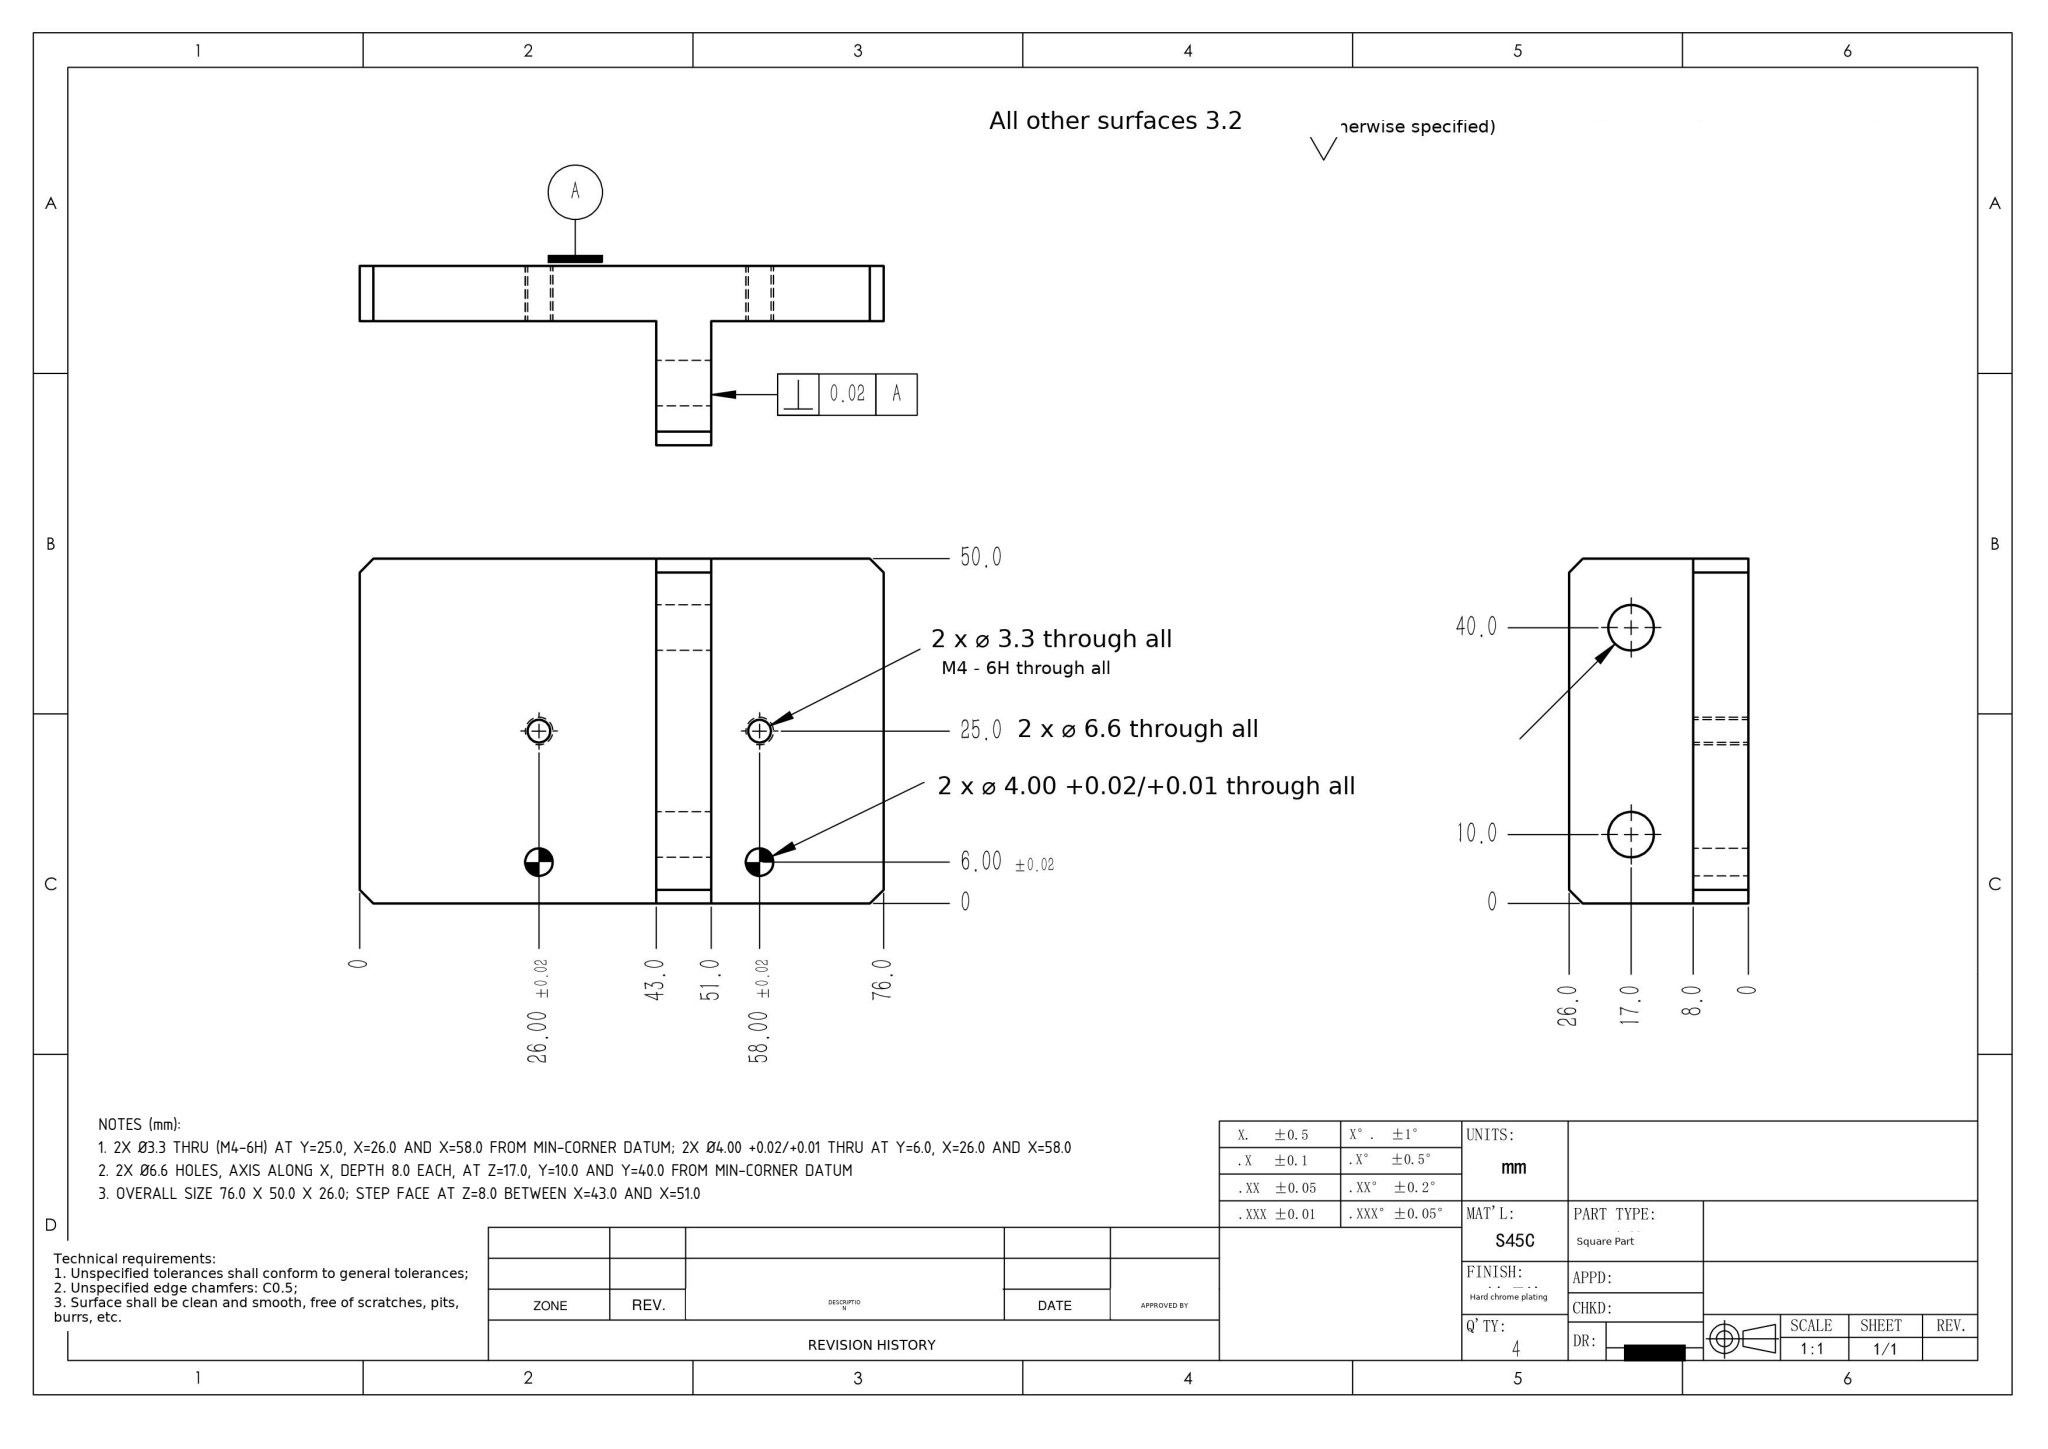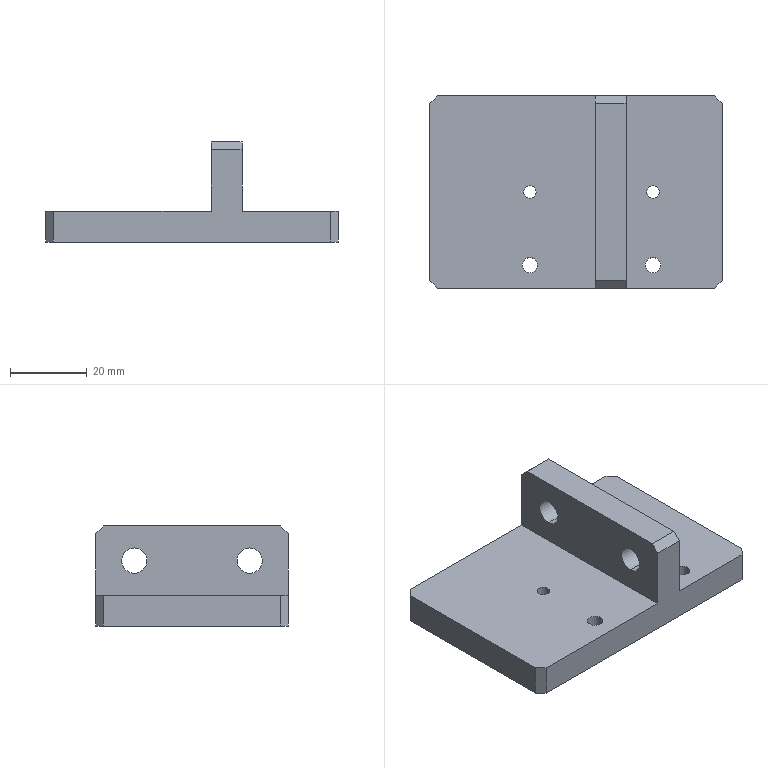Part | SolidWorks | mm | 1 solid | 28 faces | box 76 x 50 x 26 mm | volume 36619 mm3 | plane 16 | cylinder 12 | commonest cylinder face diameters 6.6 x4 4 x4 3.3 x4
Drawing notes:
2X Ø3.3 THRU (M4-6H) AT Y=25.0, X=26.0 AND X=58.0 FROM MIN-CORNER DATUM; 2X Ø4.00 +0.02/+0.01 THRU AT Y=6.0, X=26.0 AND X=58.0 | from the solid: cylinders dia 3.3 axis z at (26,25) and (58,25); dia 4.0 axis z at (26,6) and (58,6)
2X Ø6.6 HOLES, AXIS ALONG X, DEPTH 8.0 EACH, AT Z=17.0, Y=10.0 AND Y=40.0 FROM MIN-CORNER DATUM | from the solid: cylinders dia 6.6 axis x, pos (y=10,z=17) and (y=40,z=17), length 8.0
OVERALL SIZE 76.0 X 50.0 X 26.0; STEP FACE AT Z=8.0 BETWEEN X=43.0 AND X=51.0 | from the solid: bbox_xyz 76/50/26; axis_planes z=8.0 (2), x=43.0, x=51.0
build123d program:
from build123d import *

# Parameters (mm, degrees)
SKETCH1_W                 = 76
SKETCH1_H                 = 50
BOSS_EXTRUDE1_DEPTH       = 8
SKETCH2_W                 = 8
SKETCH2_H                 = 50
BOSS_EXTRUDE2_DEPTH       = 18
M4_TAPPED_HOLE1_D         = 3.3
SIZE_MM_DOWEL_PIN_HOLE1_D = 4
M6_CLEARANCE_HOLE1_D      = 6.6
CHAMFER1_SIZE             = 2


with BuildPart() as part:
    # Sketch1 → Boss-Extrude1 (new body)
    with BuildSketch(Plane.XY):
        Rectangle(SKETCH1_W, SKETCH1_H)
    extrude(amount=BOSS_EXTRUDE1_DEPTH)

    # Sketch2 → Boss-Extrude2 (add)
    with BuildSketch(Plane.XY.offset(8)):
        with Locations((9, 0)):
            Rectangle(SKETCH2_W, SKETCH2_H)
    extrude(amount=BOSS_EXTRUDE2_DEPTH)

    # M4 Tapped Hole1 (through all)
    with Locations(Plane.XY.offset(8)):
        with Locations((-12, 0), (20, 0)):
            Hole(M4_TAPPED_HOLE1_D / 2)

    # Size mm Dowel Pin Hole1 (through all)
    with Locations(Plane(origin=(0, 0, 0), x_dir=(1, 0, 0), z_dir=(0, 0, -1))):
        with Locations((-12, 19), (20, 19)):
            Hole(SIZE_MM_DOWEL_PIN_HOLE1_D / 2)

    # M6 Clearance Hole1 (through all)
    with Locations(Plane(origin=(13, 0, 0), x_dir=(0, 0, -1), z_dir=(1, 0, 0))):
        with Locations((-17, 15), (-17, -15)):
            Hole(M6_CLEARANCE_HOLE1_D / 2)

    # Chamfer1
    chamfer1_edges = [part.edges().sort_by_distance(p)[0] for p in [
        (9, -25, 26),
        (9, 25, 26),
        (38, -25, 4),
        (-38, -25, 4),
        (-38, 25, 4),
        (38, 25, 4),
    ]]
    chamfer(chamfer1_edges, length=CHAMFER1_SIZE)


solid = part.part
STEP:
#1=CARTESIAN_POINT('',(5.,15.,20.3));
#2=VERTEX_POINT('',#1);
#3=CARTESIAN_POINT('',(5.,15.,13.7));
#4=VERTEX_POINT('',#3);
#5=CARTESIAN_POINT('',(5.,15.,17.));
#6=DIRECTION('',(1.,0.,0.));
#7=DIRECTION('',(0.,1.,0.));
#8=AXIS2_PLACEMENT_3D('',#5,#6,#7);
#9=CIRCLE('',#8,3.3);
#10=EDGE_CURVE('',#2,#4,#9,.T.);
#11=ORIENTED_EDGE('',*,*,#10,.F.);
#12=CARTESIAN_POINT('',(13.,15.,20.3));
#13=VERTEX_POINT('',#12);
#14=CARTESIAN_POINT('',(13.,15.,20.3));
#15=DIRECTION('',(1.,0.,0.));
#16=VECTOR('',#15,1000.);
#17=LINE('',#14,#16);
#18=EDGE_CURVE('',#2,#13,#17,.T.);
#19=ORIENTED_EDGE('',*,*,#18,.T.);
#20=CARTESIAN_POINT('',(13.,15.,13.7));
#21=VERTEX_POINT('',#20);
#22=CARTESIAN_POINT('',(13.,15.,17.));
#23=DIRECTION('',(1.,0.,0.));
#24=DIRECTION('',(0.,0.,-1.));
#25=AXIS2_PLACEMENT_3D('',#22,#23,#24);
#26=CIRCLE('',#25,3.3);
#27=EDGE_CURVE('',#13,#21,#26,.T.);
#28=ORIENTED_EDGE('',*,*,#27,.T.);
#29=CARTESIAN_POINT('',(13.,15.,13.7));
#30=DIRECTION('',(1.,0.,0.));
#31=VECTOR('',#30,1000.);
#32=LINE('',#29,#31);
#33=EDGE_CURVE('',#4,#21,#32,.T.);
#34=ORIENTED_EDGE('',*,*,#33,.F.);
#35=EDGE_LOOP('',(#11,#19,#28,#34));
#36=FACE_OUTER_BOUND('',#35,.T.);
#37=CARTESIAN_POINT('',(13.,15.,17.));
#38=DIRECTION('',(1.,0.,0.));
#39=DIRECTION('',(0.,0.,-1.));
#40=AXIS2_PLACEMENT_3D('',#37,#38,#39);
#41=CYLINDRICAL_SURFACE('',#40,3.3);
#42=ADVANCED_FACE('',(#36),#41,.F.);
#43=CARTESIAN_POINT('',(5.,-15.,20.3));
#44=VERTEX_POINT('',#43);
#45=CARTESIAN_POINT('',(5.,-15.,13.7));
#46=VERTEX_POINT('',#45);
#47=CARTESIAN_POINT('',(5.,-15.,17.));
#48=DIRECTION('',(1.,0.,0.));
#49=DIRECTION('',(0.,1.,0.));
#50=AXIS2_PLACEMENT_3D('',#47,#48,#49);
#51=CIRCLE('',#50,3.3);
#52=EDGE_CURVE('',#44,#46,#51,.T.);
#53=ORIENTED_EDGE('',*,*,#52,.F.);
#54=CARTESIAN_POINT('',(13.,-15.,20.3));
#55=VERTEX_POINT('',#54);
#56=CARTESIAN_POINT('',(13.,-15.,20.3));
#57=DIRECTION('',(1.,0.,0.));
#58=VECTOR('',#57,1000.);
#59=LINE('',#56,#58);
#60=EDGE_CURVE('',#44,#55,#59,.T.);
#61=ORIENTED_EDGE('',*,*,#60,.T.);
#62=CARTESIAN_POINT('',(13.,-15.,13.7));
#63=VERTEX_POINT('',#62);
#64=CARTESIAN_POINT('',(13.,-15.,17.));
#65=DIRECTION('',(1.,0.,0.));
#66=DIRECTION('',(0.,0.,-1.));
#67=AXIS2_PLACEMENT_3D('',#64,#65,#66);
#68=CIRCLE('',#67,3.3);
#69=EDGE_CURVE('',#55,#63,#68,.T.);
#70=ORIENTED_EDGE('',*,*,#69,.T.);
#71=CARTESIAN_POINT('',(13.,-15.,13.7));
#72=DIRECTION('',(1.,0.,0.));
#73=VECTOR('',#72,1000.);
#74=LINE('',#71,#73);
#75=EDGE_CURVE('',#46,#63,#74,.T.);
#76=ORIENTED_EDGE('',*,*,#75,.F.);
#77=EDGE_LOOP('',(#53,#61,#70,#76));
#78=FACE_OUTER_BOUND('',#77,.T.);
#79=CARTESIAN_POINT('',(13.,-15.,17.));
#80=DIRECTION('',(1.,0.,0.));
#81=DIRECTION('',(0.,0.,-1.));
#82=AXIS2_PLACEMENT_3D('',#79,#80,#81);
#83=CYLINDRICAL_SURFACE('',#82,3.3);
#84=ADVANCED_FACE('',(#78),#83,.F.);
#85=CARTESIAN_POINT('',(-14.,-19.,8.));
#86=VERTEX_POINT('',#85);
#87=CARTESIAN_POINT('',(-10.,-19.,8.));
#88=VERTEX_POINT('',#87);
#89=CARTESIAN_POINT('',(-12.,-19.,8.));
#90=DIRECTION('',(0.,0.,1.));
#91=DIRECTION('',(1.,0.,0.));
#92=AXIS2_PLACEMENT_3D('',#89,#90,#91);
#93=CIRCLE('',#92,2.);
#94=EDGE_CURVE('',#86,#88,#93,.T.);
#95=ORIENTED_EDGE('',*,*,#94,.T.);
#96=CARTESIAN_POINT('',(-10.,-19.,0.));
#97=VERTEX_POINT('',#96);
#98=CARTESIAN_POINT('',(-10.,-19.,0.));
#99=DIRECTION('',(0.,0.,-1.));
#100=VECTOR('',#99,1000.);
#101=LINE('',#98,#100);
#102=EDGE_CURVE('',#88,#97,#101,.T.);
#103=ORIENTED_EDGE('',*,*,#102,.T.);
#104=CARTESIAN_POINT('',(-14.,-19.,0.));
#105=VERTEX_POINT('',#104);
#106=CARTESIAN_POINT('',(-12.,-19.,0.));
#107=DIRECTION('',(0.,0.,-1.));
#108=DIRECTION('',(-1.,0.,0.));
#109=AXIS2_PLACEMENT_3D('',#106,#107,#108);
#110=CIRCLE('',#109,2.);
#111=EDGE_CURVE('',#97,#105,#110,.T.);
#112=ORIENTED_EDGE('',*,*,#111,.T.);
#113=CARTESIAN_POINT('',(-14.,-19.,0.));
#114=DIRECTION('',(0.,0.,-1.));
#115=VECTOR('',#114,1000.);
#116=LINE('',#113,#115);
#117=EDGE_CURVE('',#86,#105,#116,.T.);
#118=ORIENTED_EDGE('',*,*,#117,.F.);
#119=EDGE_LOOP('',(#95,#103,#112,#118));
#120=FACE_OUTER_BOUND('',#119,.T.);
#121=CARTESIAN_POINT('',(-12.,-19.,0.));
#122=DIRECTION('',(0.,0.,-1.));
#123=DIRECTION('',(-1.,0.,0.));
#124=AXIS2_PLACEMENT_3D('',#121,#122,#123);
#125=CYLINDRICAL_SURFACE('',#124,2.);
#126=ADVANCED_FACE('',(#120),#125,.F.);
#127=CARTESIAN_POINT('',(18.,-19.,8.));
#128=VERTEX_POINT('',#127);
#129=CARTESIAN_POINT('',(22.,-19.,8.));
#130=VERTEX_POINT('',#129);
#131=CARTESIAN_POINT('',(20.,-19.,8.));
#132=DIRECTION('',(0.,0.,1.));
#133=DIRECTION('',(1.,0.,0.));
#134=AXIS2_PLACEMENT_3D('',#131,#132,#133);
#135=CIRCLE('',#134,2.);
#136=EDGE_CURVE('',#128,#130,#135,.T.);
#137=ORIENTED_EDGE('',*,*,#136,.T.);
#138=CARTESIAN_POINT('',(22.,-19.,0.));
#139=VERTEX_POINT('',#138);
#140=CARTESIAN_POINT('',(22.,-19.,0.));
#141=DIRECTION('',(0.,0.,-1.));
#142=VECTOR('',#141,1000.);
#143=LINE('',#140,#142);
#144=EDGE_CURVE('',#130,#139,#143,.T.);
#145=ORIENTED_EDGE('',*,*,#144,.T.);
#146=CARTESIAN_POINT('',(18.,-19.,0.));
#147=VERTEX_POINT('',#146);
#148=CARTESIAN_POINT('',(20.,-19.,0.));
#149=DIRECTION('',(0.,0.,-1.));
#150=DIRECTION('',(-1.,0.,0.));
#151=AXIS2_PLACEMENT_3D('',#148,#149,#150);
#152=CIRCLE('',#151,2.);
#153=EDGE_CURVE('',#139,#147,#152,.T.);
#154=ORIENTED_EDGE('',*,*,#153,.T.);
#155=CARTESIAN_POINT('',(18.,-19.,0.));
#156=DIRECTION('',(0.,0.,-1.));
#157=VECTOR('',#156,1000.);
#158=LINE('',#155,#157);
#159=EDGE_CURVE('',#128,#147,#158,.T.);
#160=ORIENTED_EDGE('',*,*,#159,.F.);
#161=EDGE_LOOP('',(#137,#145,#154,#160));
#162=FACE_OUTER_BOUND('',#161,.T.);
#163=CARTESIAN_POINT('',(20.,-19.,0.));
#164=DIRECTION('',(0.,0.,-1.));
#165=DIRECTION('',(-1.,0.,0.));
#166=AXIS2_PLACEMENT_3D('',#163,#164,#165);
#167=CYLINDRICAL_SURFACE('',#166,2.);
#168=ADVANCED_FACE('',(#162),#167,.F.);
#169=CARTESIAN_POINT('',(-13.65,0.,0.));
#170=VERTEX_POINT('',#169);
#171=CARTESIAN_POINT('',(-10.35,0.,0.));
#172=VERTEX_POINT('',#171);
#173=CARTESIAN_POINT('',(-12.,0.,0.));
#174=DIRECTION('',(0.,0.,1.));
#175=DIRECTION('',(1.,0.,0.));
#176=AXIS2_PLACEMENT_3D('',#173,#174,#175);
#177=CIRCLE('',#176,1.65);
#178=EDGE_CURVE('',#170,#172,#177,.T.);
#179=ORIENTED_EDGE('',*,*,#178,.F.);
#180=CARTESIAN_POINT('',(-13.65,0.,8.));
#181=VERTEX_POINT('',#180);
#182=CARTESIAN_POINT('',(-13.65,0.,8.));
#183=DIRECTION('',(0.,0.,1.));
#184=VECTOR('',#183,1000.);
#185=LINE('',#182,#184);
#186=EDGE_CURVE('',#170,#181,#185,.T.);
#187=ORIENTED_EDGE('',*,*,#186,.T.);
#188=CARTESIAN_POINT('',(-10.35,0.,8.));
#189=VERTEX_POINT('',#188);
#190=CARTESIAN_POINT('',(-12.,0.,8.));
#191=DIRECTION('',(0.,0.,1.));
#192=DIRECTION('',(1.,0.,0.));
#193=AXIS2_PLACEMENT_3D('',#190,#191,#192);
#194=CIRCLE('',#193,1.65);
#195=EDGE_CURVE('',#181,#189,#194,.T.);
#196=ORIENTED_EDGE('',*,*,#195,.T.);
#197=CARTESIAN_POINT('',(-10.35,0.,8.));
#198=DIRECTION('',(0.,0.,1.));
#199=VECTOR('',#198,1000.);
#200=LINE('',#197,#199);
#201=EDGE_CURVE('',#172,#189,#200,.T.);
#202=ORIENTED_EDGE('',*,*,#201,.F.);
#203=EDGE_LOOP('',(#179,#187,#196,#202));
#204=FACE_OUTER_BOUND('',#203,.T.);
#205=CARTESIAN_POINT('',(-12.,0.,8.));
#206=DIRECTION('',(0.,0.,1.));
#207=DIRECTION('',(1.,0.,0.));
#208=AXIS2_PLACEMENT_3D('',#205,#206,#207);
#209=CYLINDRICAL_SURFACE('',#208,1.65);
#210=ADVANCED_FACE('',(#204),#209,.F.);
#211=CARTESIAN_POINT('',(18.35,0.,0.));
#212=VERTEX_POINT('',#211);
#213=CARTESIAN_POINT('',(21.65,0.,0.));
#214=VERTEX_POINT('',#213);
#215=CARTESIAN_POINT('',(20.,0.,0.));
#216=DIRECTION('',(0.,0.,1.));
#217=DIRECTION('',(1.,0.,0.));
#218=AXIS2_PLACEMENT_3D('',#215,#216,#217);
#219=CIRCLE('',#218,1.65);
#220=EDGE_CURVE('',#212,#214,#219,.T.);
#221=ORIENTED_EDGE('',*,*,#220,.F.);
#222=CARTESIAN_POINT('',(18.35,0.,8.));
#223=VERTEX_POINT('',#222);
#224=CARTESIAN_POINT('',(18.35,0.,8.));
#225=DIRECTION('',(0.,0.,1.));
#226=VECTOR('',#225,1000.);
#227=LINE('',#224,#226);
#228=EDGE_CURVE('',#212,#223,#227,.T.);
#229=ORIENTED_EDGE('',*,*,#228,.T.);
#230=CARTESIAN_POINT('',(21.65,0.,8.));
#231=VERTEX_POINT('',#230);
#232=CARTESIAN_POINT('',(20.,0.,8.));
#233=DIRECTION('',(0.,0.,1.));
#234=DIRECTION('',(1.,0.,0.));
#235=AXIS2_PLACEMENT_3D('',#232,#233,#234);
#236=CIRCLE('',#235,1.65);
#237=EDGE_CURVE('',#223,#231,#236,.T.);
#238=ORIENTED_EDGE('',*,*,#237,.T.);
#239=CARTESIAN_POINT('',(21.65,0.,8.));
#240=DIRECTION('',(0.,0.,1.));
#241=VECTOR('',#240,1000.);
#242=LINE('',#239,#241);
#243=EDGE_CURVE('',#214,#231,#242,.T.);
#244=ORIENTED_EDGE('',*,*,#243,.F.);
#245=EDGE_LOOP('',(#221,#229,#238,#244));
#246=FACE_OUTER_BOUND('',#245,.T.);
#247=CARTESIAN_POINT('',(20.,0.,8.));
#248=DIRECTION('',(0.,0.,1.));
#249=DIRECTION('',(1.,0.,0.));
#250=AXIS2_PLACEMENT_3D('',#247,#248,#249);
#251=CYLINDRICAL_SURFACE('',#250,1.65);
#252=ADVANCED_FACE('',(#246),#251,.F.);
#253=ORIENTED_EDGE('',*,*,#94,.F.);
#254=CARTESIAN_POINT('',(-12.,-19.,8.));
#255=DIRECTION('',(0.,0.,1.));
#256=DIRECTION('',(1.,0.,0.));
#257=AXIS2_PLACEMENT_3D('',#254,#255,#256);
#258=CIRCLE('',#257,2.);
#259=EDGE_CURVE('',#88,#86,#258,.T.);
#260=ORIENTED_EDGE('',*,*,#259,.F.);
#261=EDGE_LOOP('',(#253,#260));
#262=FACE_BOUND('',#261,.T.);
#263=CARTESIAN_POINT('',(-12.,0.,8.));
#264=DIRECTION('',(0.,0.,1.));
#265=DIRECTION('',(1.,0.,0.));
#266=AXIS2_PLACEMENT_3D('',#263,#264,#265);
#267=CIRCLE('',#266,1.65);
#268=EDGE_CURVE('',#189,#181,#267,.T.);
#269=ORIENTED_EDGE('',*,*,#268,.F.);
#270=ORIENTED_EDGE('',*,*,#195,.F.);
#271=EDGE_LOOP('',(#269,#270));
#272=FACE_BOUND('',#271,.T.);
#273=CARTESIAN_POINT('',(5.,25.,8.));
#274=VERTEX_POINT('',#273);
#275=CARTESIAN_POINT('',(-36.,25.,8.));
#276=VERTEX_POINT('',#275);
#277=CARTESIAN_POINT('',(-38.,25.,8.));
#278=DIRECTION('',(-1.,0.,0.));
#279=VECTOR('',#278,1000.);
#280=LINE('',#277,#279);
#281=EDGE_CURVE('',#274,#276,#280,.T.);
#282=ORIENTED_EDGE('',*,*,#281,.T.);
#283=CARTESIAN_POINT('',(-38.,23.,8.));
#284=VERTEX_POINT('',#283);
#285=CARTESIAN_POINT('',(-30.5,30.5,8.));
#286=DIRECTION('',(-0.7071,-0.7071,0.));
#287=VECTOR('',#286,1000.);
#288=LINE('',#285,#287);
#289=EDGE_CURVE('',#276,#284,#288,.T.);
#290=ORIENTED_EDGE('',*,*,#289,.T.);
#291=CARTESIAN_POINT('',(-38.,-23.,8.));
#292=VERTEX_POINT('',#291);
#293=CARTESIAN_POINT('',(-38.,25.,8.));
#294=DIRECTION('',(0.,-1.,0.));
#295=VECTOR('',#294,1000.);
#296=LINE('',#293,#295);
#297=EDGE_CURVE('',#284,#292,#296,.T.);
#298=ORIENTED_EDGE('',*,*,#297,.T.);
#299=CARTESIAN_POINT('',(-36.,-25.,8.));
#300=VERTEX_POINT('',#299);
#301=CARTESIAN_POINT('',(-30.5,-30.5,8.));
#302=DIRECTION('',(0.7071,-0.7071,0.));
#303=VECTOR('',#302,1000.);
#304=LINE('',#301,#303);
#305=EDGE_CURVE('',#292,#300,#304,.T.);
#306=ORIENTED_EDGE('',*,*,#305,.T.);
#307=CARTESIAN_POINT('',(5.,-25.,8.));
#308=VERTEX_POINT('',#307);
#309=CARTESIAN_POINT('',(-38.,-25.,8.));
#310=DIRECTION('',(1.,0.,0.));
#311=VECTOR('',#310,1000.);
#312=LINE('',#309,#311);
#313=EDGE_CURVE('',#300,#308,#312,.T.);
#314=ORIENTED_EDGE('',*,*,#313,.T.);
#315=CARTESIAN_POINT('',(5.,25.,8.));
#316=DIRECTION('',(0.,-1.,0.));
#317=VECTOR('',#316,1000.);
#318=LINE('',#315,#317);
#319=EDGE_CURVE('',#274,#308,#318,.T.);
#320=ORIENTED_EDGE('',*,*,#319,.F.);
#321=EDGE_LOOP('',(#282,#290,#298,#306,#314,#320));
#322=FACE_OUTER_BOUND('',#321,.T.);
#323=CARTESIAN_POINT('',(0.,0.,8.));
#324=DIRECTION('',(0.,0.,1.));
#325=DIRECTION('',(1.,0.,0.));
#326=AXIS2_PLACEMENT_3D('',#323,#324,#325);
#327=PLANE('',#326);
#328=ADVANCED_FACE('',(#262,#272,#322),#327,.T.);
#329=CARTESIAN_POINT('',(38.,-23.,8.));
#330=VERTEX_POINT('',#329);
#331=CARTESIAN_POINT('',(38.,23.,8.));
#332=VERTEX_POINT('',#331);
#333=CARTESIAN_POINT('',(38.,25.,8.));
#334=DIRECTION('',(-0.,1.,0.));
#335=VECTOR('',#334,1000.);
#336=LINE('',#333,#335);
#337=EDGE_CURVE('',#330,#332,#336,.T.);
#338=ORIENTED_EDGE('',*,*,#337,.F.);
#339=CARTESIAN_POINT('',(38.,-23.,0.));
#340=VERTEX_POINT('',#339);
#341=CARTESIAN_POINT('',(38.,-23.,8.));
#342=DIRECTION('',(0.,0.,-1.));
#343=VECTOR('',#342,1000.);
#344=LINE('',#341,#343);
#345=EDGE_CURVE('',#330,#340,#344,.T.);
#346=ORIENTED_EDGE('',*,*,#345,.T.);
#347=CARTESIAN_POINT('',(38.,23.,0.));
#348=VERTEX_POINT('',#347);
#349=CARTESIAN_POINT('',(38.,25.,0.));
#350=DIRECTION('',(-0.,1.,0.));
#351=VECTOR('',#350,1000.);
#352=LINE('',#349,#351);
#353=EDGE_CURVE('',#340,#348,#352,.T.);
#354=ORIENTED_EDGE('',*,*,#353,.T.);
#355=CARTESIAN_POINT('',(38.,23.,8.));
#356=DIRECTION('',(0.,0.,1.));
#357=VECTOR('',#356,1000.);
#358=LINE('',#355,#357);
#359=EDGE_CURVE('',#348,#332,#358,.T.);
#360=ORIENTED_EDGE('',*,*,#359,.T.);
#361=EDGE_LOOP('',(#338,#346,#354,#360));
#362=FACE_OUTER_BOUND('',#361,.T.);
#363=CARTESIAN_POINT('',(38.,25.,8.));
#364=DIRECTION('',(-1.,-0.,0.));
#365=DIRECTION('',(0.,-1.,0.));
#366=AXIS2_PLACEMENT_3D('',#363,#364,#365);
#367=PLANE('',#366);
#368=ADVANCED_FACE('',(#362),#367,.F.);
#369=CARTESIAN_POINT('',(36.,25.,8.));
#370=VERTEX_POINT('',#369);
#371=CARTESIAN_POINT('',(13.,25.,8.));
#372=VERTEX_POINT('',#371);
#373=CARTESIAN_POINT('',(-38.,25.,8.));
#374=DIRECTION('',(-1.,0.,0.));
#375=VECTOR('',#374,1000.);
#376=LINE('',#373,#375);
#377=EDGE_CURVE('',#370,#372,#376,.T.);
#378=ORIENTED_EDGE('',*,*,#377,.F.);
#379=CARTESIAN_POINT('',(36.,25.,0.));
#380=VERTEX_POINT('',#379);
#381=CARTESIAN_POINT('',(36.,25.,8.));
#382=DIRECTION('',(0.,0.,-1.));
#383=VECTOR('',#382,1000.);
#384=LINE('',#381,#383);
#385=EDGE_CURVE('',#370,#380,#384,.T.);
#386=ORIENTED_EDGE('',*,*,#385,.T.);
#387=CARTESIAN_POINT('',(-36.,25.,0.));
#388=VERTEX_POINT('',#387);
#389=CARTESIAN_POINT('',(-38.,25.,0.));
#390=DIRECTION('',(-1.,0.,0.));
#391=VECTOR('',#390,1000.);
#392=LINE('',#389,#391);
#393=EDGE_CURVE('',#380,#388,#392,.T.);
#394=ORIENTED_EDGE('',*,*,#393,.T.);
#395=CARTESIAN_POINT('',(-36.,25.,8.));
#396=DIRECTION('',(0.,0.,1.));
#397=VECTOR('',#396,1000.);
#398=LINE('',#395,#397);
#399=EDGE_CURVE('',#388,#276,#398,.T.);
#400=ORIENTED_EDGE('',*,*,#399,.T.);
#401=ORIENTED_EDGE('',*,*,#281,.F.);
#402=CARTESIAN_POINT('',(5.,25.,24.));
#403=VERTEX_POINT('',#402);
#404=CARTESIAN_POINT('',(5.,25.,26.));
#405=DIRECTION('',(0.,0.,-1.));
#406=VECTOR('',#405,1000.);
#407=LINE('',#404,#406);
#408=EDGE_CURVE('',#403,#274,#407,.T.);
#409=ORIENTED_EDGE('',*,*,#408,.F.);
#410=CARTESIAN_POINT('',(13.,25.,24.));
#411=VERTEX_POINT('',#410);
#412=CARTESIAN_POINT('',(13.,25.,24.));
#413=DIRECTION('',(1.,0.,0.));
#414=VECTOR('',#413,1000.);
#415=LINE('',#412,#414);
#416=EDGE_CURVE('',#403,#411,#415,.T.);
#417=ORIENTED_EDGE('',*,*,#416,.T.);
#418=CARTESIAN_POINT('',(13.,25.,26.));
#419=DIRECTION('',(0.,0.,-1.));
#420=VECTOR('',#419,1000.);
#421=LINE('',#418,#420);
#422=EDGE_CURVE('',#411,#372,#421,.T.);
#423=ORIENTED_EDGE('',*,*,#422,.T.);
#424=EDGE_LOOP('',(#378,#386,#394,#400,#401,#409,#417,#423));
#425=FACE_OUTER_BOUND('',#424,.T.);
#426=CARTESIAN_POINT('',(-38.,25.,8.));
#427=DIRECTION('',(0.,-1.,0.));
#428=DIRECTION('',(0.,0.,-1.));
#429=AXIS2_PLACEMENT_3D('',#426,#427,#428);
#430=PLANE('',#429);
#431=ADVANCED_FACE('',(#425),#430,.F.);
#432=ORIENTED_EDGE('',*,*,#297,.F.);
#433=CARTESIAN_POINT('',(-38.,23.,0.));
#434=VERTEX_POINT('',#433);
#435=CARTESIAN_POINT('',(-38.,23.,8.));
#436=DIRECTION('',(0.,0.,-1.));
#437=VECTOR('',#436,1000.);
#438=LINE('',#435,#437);
#439=EDGE_CURVE('',#284,#434,#438,.T.);
#440=ORIENTED_EDGE('',*,*,#439,.T.);
#441=CARTESIAN_POINT('',(-38.,-23.,0.));
#442=VERTEX_POINT('',#441);
#443=CARTESIAN_POINT('',(-38.,25.,0.));
#444=DIRECTION('',(0.,-1.,0.));
#445=VECTOR('',#444,1000.);
#446=LINE('',#443,#445);
#447=EDGE_CURVE('',#434,#442,#446,.T.);
#448=ORIENTED_EDGE('',*,*,#447,.T.);
#449=CARTESIAN_POINT('',(-38.,-23.,8.));
#450=DIRECTION('',(0.,0.,1.));
#451=VECTOR('',#450,1000.);
#452=LINE('',#449,#451);
#453=EDGE_CURVE('',#442,#292,#452,.T.);
#454=ORIENTED_EDGE('',*,*,#453,.T.);
#455=EDGE_LOOP('',(#432,#440,#448,#454));
#456=FACE_OUTER_BOUND('',#455,.T.);
#457=CARTESIAN_POINT('',(-38.,25.,8.));
#458=DIRECTION('',(1.,0.,0.));
#459=DIRECTION('',(-0.,1.,0.));
#460=AXIS2_PLACEMENT_3D('',#457,#458,#459);
#461=PLANE('',#460);
#462=ADVANCED_FACE('',(#456),#461,.F.);
#463=CARTESIAN_POINT('',(-36.,-25.,0.));
#464=VERTEX_POINT('',#463);
#465=CARTESIAN_POINT('',(36.,-25.,0.));
#466=VERTEX_POINT('',#465);
#467=CARTESIAN_POINT('',(-38.,-25.,0.));
#468=DIRECTION('',(1.,0.,0.));
#469=VECTOR('',#468,1000.);
#470=LINE('',#467,#469);
#471=EDGE_CURVE('',#464,#466,#470,.T.);
#472=ORIENTED_EDGE('',*,*,#471,.T.);
#473=CARTESIAN_POINT('',(36.,-25.,8.));
#474=VERTEX_POINT('',#473);
#475=CARTESIAN_POINT('',(36.,-25.,8.));
#476=DIRECTION('',(0.,0.,1.));
#477=VECTOR('',#476,1000.);
#478=LINE('',#475,#477);
#479=EDGE_CURVE('',#466,#474,#478,.T.);
#480=ORIENTED_EDGE('',*,*,#479,.T.);
#481=CARTESIAN_POINT('',(13.,-25.,8.));
#482=VERTEX_POINT('',#481);
#483=CARTESIAN_POINT('',(-38.,-25.,8.));
#484=DIRECTION('',(1.,0.,0.));
#485=VECTOR('',#484,1000.);
#486=LINE('',#483,#485);
#487=EDGE_CURVE('',#482,#474,#486,.T.);
#488=ORIENTED_EDGE('',*,*,#487,.F.);
#489=CARTESIAN_POINT('',(13.,-25.,24.));
#490=VERTEX_POINT('',#489);
#491=CARTESIAN_POINT('',(13.,-25.,26.));
#492=DIRECTION('',(0.,0.,-1.));
#493=VECTOR('',#492,1000.);
#494=LINE('',#491,#493);
#495=EDGE_CURVE('',#490,#482,#494,.T.);
#496=ORIENTED_EDGE('',*,*,#495,.F.);
#497=CARTESIAN_POINT('',(5.,-25.,24.));
#498=VERTEX_POINT('',#497);
#499=CARTESIAN_POINT('',(5.,-25.,24.));
#500=DIRECTION('',(-1.,0.,0.));
#501=VECTOR('',#500,1000.);
#502=LINE('',#499,#501);
#503=EDGE_CURVE('',#490,#498,#502,.T.);
#504=ORIENTED_EDGE('',*,*,#503,.T.);
#505=CARTESIAN_POINT('',(5.,-25.,26.));
#506=DIRECTION('',(0.,0.,-1.));
#507=VECTOR('',#506,1000.);
#508=LINE('',#505,#507);
#509=EDGE_CURVE('',#498,#308,#508,.T.);
#510=ORIENTED_EDGE('',*,*,#509,.T.);
#511=ORIENTED_EDGE('',*,*,#313,.F.);
#512=CARTESIAN_POINT('',(-36.,-25.,8.));
#513=DIRECTION('',(0.,0.,-1.));
#514=VECTOR('',#513,1000.);
#515=LINE('',#512,#514);
#516=EDGE_CURVE('',#300,#464,#515,.T.);
#517=ORIENTED_EDGE('',*,*,#516,.T.);
#518=EDGE_LOOP('',(#472,#480,#488,#496,#504,#510,#511,#517));
#519=FACE_OUTER_BOUND('',#518,.T.);
#520=CARTESIAN_POINT('',(-38.,-25.,8.));
#521=DIRECTION('',(0.,1.,0.));
#522=DIRECTION('',(0.,0.,1.));
#523=AXIS2_PLACEMENT_3D('',#520,#521,#522);
#524=PLANE('',#523);
#525=ADVANCED_FACE('',(#519),#524,.F.);
#526=ORIENTED_EDGE('',*,*,#136,.F.);
#527=CARTESIAN_POINT('',(20.,-19.,8.));
#528=DIRECTION('',(0.,0.,1.));
#529=DIRECTION('',(1.,0.,0.));
#530=AXIS2_PLACEMENT_3D('',#527,#528,#529);
#531=CIRCLE('',#530,2.);
#532=EDGE_CURVE('',#130,#128,#531,.T.);
#533=ORIENTED_EDGE('',*,*,#532,.F.);
#534=EDGE_LOOP('',(#526,#533));
#535=FACE_BOUND('',#534,.T.);
#536=CARTESIAN_POINT('',(20.,0.,8.));
#537=DIRECTION('',(0.,0.,1.));
#538=DIRECTION('',(1.,0.,0.));
#539=AXIS2_PLACEMENT_3D('',#536,#537,#538);
#540=CIRCLE('',#539,1.65);
#541=EDGE_CURVE('',#231,#223,#540,.T.);
#542=ORIENTED_EDGE('',*,*,#541,.F.);
#543=ORIENTED_EDGE('',*,*,#237,.F.);
#544=EDGE_LOOP('',(#542,#543));
#545=FACE_BOUND('',#544,.T.);
#546=ORIENTED_EDGE('',*,*,#487,.T.);
#547=CARTESIAN_POINT('',(30.5,-30.5,8.));
#548=DIRECTION('',(0.7071,0.7071,0.));
#549=VECTOR('',#548,1000.);
#550=LINE('',#547,#549);
#551=EDGE_CURVE('',#474,#330,#550,.T.);
#552=ORIENTED_EDGE('',*,*,#551,.T.);
#553=ORIENTED_EDGE('',*,*,#337,.T.);
#554=CARTESIAN_POINT('',(30.5,30.5,8.));
#555=DIRECTION('',(-0.7071,0.7071,0.));
#556=VECTOR('',#555,1000.);
#557=LINE('',#554,#556);
#558=EDGE_CURVE('',#332,#370,#557,.T.);
#559=ORIENTED_EDGE('',*,*,#558,.T.);
#560=ORIENTED_EDGE('',*,*,#377,.T.);
#561=CARTESIAN_POINT('',(13.,25.,8.));
#562=DIRECTION('',(-0.,1.,0.));
#563=VECTOR('',#562,1000.);
#564=LINE('',#561,#563);
#565=EDGE_CURVE('',#482,#372,#564,.T.);
#566=ORIENTED_EDGE('',*,*,#565,.F.);
#567=EDGE_LOOP('',(#546,#552,#553,#559,#560,#566));
#568=FACE_OUTER_BOUND('',#567,.T.);
#569=CARTESIAN_POINT('',(0.,0.,8.));
#570=DIRECTION('',(0.,0.,1.));
#571=DIRECTION('',(1.,0.,0.));
#572=AXIS2_PLACEMENT_3D('',#569,#570,#571);
#573=PLANE('',#572);
#574=ADVANCED_FACE('',(#535,#545,#568),#573,.T.);
#575=CARTESIAN_POINT('',(-12.,-19.,0.));
#576=DIRECTION('',(0.,0.,-1.));
#577=DIRECTION('',(-1.,0.,0.));
#578=AXIS2_PLACEMENT_3D('',#575,#576,#577);
#579=CIRCLE('',#578,2.);
#580=EDGE_CURVE('',#105,#97,#579,.T.);
#581=ORIENTED_EDGE('',*,*,#580,.F.);
#582=ORIENTED_EDGE('',*,*,#111,.F.);
#583=EDGE_LOOP('',(#581,#582));
#584=FACE_BOUND('',#583,.T.);
#585=CARTESIAN_POINT('',(20.,-19.,0.));
#586=DIRECTION('',(0.,0.,-1.));
#587=DIRECTION('',(-1.,0.,0.));
#588=AXIS2_PLACEMENT_3D('',#585,#586,#587);
#589=CIRCLE('',#588,2.);
#590=EDGE_CURVE('',#147,#139,#589,.T.);
#591=ORIENTED_EDGE('',*,*,#590,.F.);
#592=ORIENTED_EDGE('',*,*,#153,.F.);
#593=EDGE_LOOP('',(#591,#592));
#594=FACE_BOUND('',#593,.T.);
#595=CARTESIAN_POINT('',(-12.,0.,0.));
#596=DIRECTION('',(0.,0.,1.));
#597=DIRECTION('',(1.,0.,0.));
#598=AXIS2_PLACEMENT_3D('',#595,#596,#597);
#599=CIRCLE('',#598,1.65);
#600=EDGE_CURVE('',#172,#170,#599,.T.);
#601=ORIENTED_EDGE('',*,*,#600,.T.);
#602=ORIENTED_EDGE('',*,*,#178,.T.);
#603=EDGE_LOOP('',(#601,#602));
#604=FACE_BOUND('',#603,.T.);
#605=CARTESIAN_POINT('',(20.,0.,0.));
#606=DIRECTION('',(0.,0.,1.));
#607=DIRECTION('',(1.,0.,0.));
#608=AXIS2_PLACEMENT_3D('',#605,#606,#607);
#609=CIRCLE('',#608,1.65);
#610=EDGE_CURVE('',#214,#212,#609,.T.);
#611=ORIENTED_EDGE('',*,*,#610,.T.);
#612=ORIENTED_EDGE('',*,*,#220,.T.);
#613=EDGE_LOOP('',(#611,#612));
#614=FACE_BOUND('',#613,.T.);
#615=ORIENTED_EDGE('',*,*,#353,.F.);
#616=CARTESIAN_POINT('',(38.,-23.,0.));
#617=DIRECTION('',(-0.7071,-0.7071,0.));
#618=VECTOR('',#617,1000.);
#619=LINE('',#616,#618);
#620=EDGE_CURVE('',#340,#466,#619,.T.);
#621=ORIENTED_EDGE('',*,*,#620,.T.);
#622=ORIENTED_EDGE('',*,*,#471,.F.);
#623=CARTESIAN_POINT('',(-36.,-25.,0.));
#624=DIRECTION('',(-0.7071,0.7071,0.));
#625=VECTOR('',#624,1000.);
#626=LINE('',#623,#625);
#627=EDGE_CURVE('',#464,#442,#626,.T.);
#628=ORIENTED_EDGE('',*,*,#627,.T.);
#629=ORIENTED_EDGE('',*,*,#447,.F.);
#630=CARTESIAN_POINT('',(-38.,23.,0.));
#631=DIRECTION('',(0.7071,0.7071,0.));
#632=VECTOR('',#631,1000.);
#633=LINE('',#630,#632);
#634=EDGE_CURVE('',#434,#388,#633,.T.);
#635=ORIENTED_EDGE('',*,*,#634,.T.);
#636=ORIENTED_EDGE('',*,*,#393,.F.);
#637=CARTESIAN_POINT('',(36.,25.,0.));
#638=DIRECTION('',(0.7071,-0.7071,0.));
#639=VECTOR('',#638,1000.);
#640=LINE('',#637,#639);
#641=EDGE_CURVE('',#380,#348,#640,.T.);
#642=ORIENTED_EDGE('',*,*,#641,.T.);
#643=EDGE_LOOP('',(#615,#621,#622,#628,#629,#635,#636,#642));
#644=FACE_OUTER_BOUND('',#643,.T.);
#645=CARTESIAN_POINT('',(0.,0.,0.));
#646=DIRECTION('',(0.,0.,1.));
#647=DIRECTION('',(1.,0.,0.));
#648=AXIS2_PLACEMENT_3D('',#645,#646,#647);
#649=PLANE('',#648);
#650=ADVANCED_FACE('',(#584,#594,#604,#614,#644),#649,.F.);
#651=CARTESIAN_POINT('',(5.,15.,17.));
#652=DIRECTION('',(1.,0.,0.));
#653=DIRECTION('',(0.,1.,0.));
#654=AXIS2_PLACEMENT_3D('',#651,#652,#653);
#655=CIRCLE('',#654,3.3);
#656=EDGE_CURVE('',#4,#2,#655,.T.);
#657=ORIENTED_EDGE('',*,*,#656,.T.);
#658=ORIENTED_EDGE('',*,*,#10,.T.);
#659=EDGE_LOOP('',(#657,#658));
#660=FACE_BOUND('',#659,.T.);
#661=CARTESIAN_POINT('',(5.,-15.,17.));
#662=DIRECTION('',(1.,0.,0.));
#663=DIRECTION('',(0.,1.,0.));
#664=AXIS2_PLACEMENT_3D('',#661,#662,#663);
#665=CIRCLE('',#664,3.3);
#666=EDGE_CURVE('',#46,#44,#665,.T.);
#667=ORIENTED_EDGE('',*,*,#666,.T.);
#668=ORIENTED_EDGE('',*,*,#52,.T.);
#669=EDGE_LOOP('',(#667,#668));
#670=FACE_BOUND('',#669,.T.);
#671=CARTESIAN_POINT('',(5.,23.,26.));
#672=VERTEX_POINT('',#671);
#673=CARTESIAN_POINT('',(5.,-23.,26.));
#674=VERTEX_POINT('',#673);
#675=CARTESIAN_POINT('',(5.,25.,26.));
#676=DIRECTION('',(0.,-1.,0.));
#677=VECTOR('',#676,1000.);
#678=LINE('',#675,#677);
#679=EDGE_CURVE('',#672,#674,#678,.T.);
#680=ORIENTED_EDGE('',*,*,#679,.F.);
#681=CARTESIAN_POINT('',(5.,23.,26.));
#682=DIRECTION('',(-0.,0.7071,-0.7071));
#683=VECTOR('',#682,1000.);
#684=LINE('',#681,#683);
#685=EDGE_CURVE('',#672,#403,#684,.T.);
#686=ORIENTED_EDGE('',*,*,#685,.T.);
#687=ORIENTED_EDGE('',*,*,#408,.T.);
#688=ORIENTED_EDGE('',*,*,#319,.T.);
#689=ORIENTED_EDGE('',*,*,#509,.F.);
#690=CARTESIAN_POINT('',(5.,-23.,26.));
#691=DIRECTION('',(-0.,0.7071,0.7071));
#692=VECTOR('',#691,1000.);
#693=LINE('',#690,#692);
#694=EDGE_CURVE('',#498,#674,#693,.T.);
#695=ORIENTED_EDGE('',*,*,#694,.T.);
#696=EDGE_LOOP('',(#680,#686,#687,#688,#689,#695));
#697=FACE_OUTER_BOUND('',#696,.T.);
#698=CARTESIAN_POINT('',(5.,25.,26.));
#699=DIRECTION('',(1.,0.,0.));
#700=DIRECTION('',(-0.,1.,0.));
#701=AXIS2_PLACEMENT_3D('',#698,#699,#700);
#702=PLANE('',#701);
#703=ADVANCED_FACE('',(#660,#670,#697),#702,.F.);
#704=CARTESIAN_POINT('',(13.,15.,17.));
#705=DIRECTION('',(1.,0.,0.));
#706=DIRECTION('',(0.,0.,-1.));
#707=AXIS2_PLACEMENT_3D('',#704,#705,#706);
#708=CIRCLE('',#707,3.3);
#709=EDGE_CURVE('',#21,#13,#708,.T.);
#710=ORIENTED_EDGE('',*,*,#709,.F.);
#711=ORIENTED_EDGE('',*,*,#27,.F.);
#712=EDGE_LOOP('',(#710,#711));
#713=FACE_BOUND('',#712,.T.);
#714=CARTESIAN_POINT('',(13.,-15.,17.));
#715=DIRECTION('',(1.,0.,0.));
#716=DIRECTION('',(0.,0.,-1.));
#717=AXIS2_PLACEMENT_3D('',#714,#715,#716);
#718=CIRCLE('',#717,3.3);
#719=EDGE_CURVE('',#63,#55,#718,.T.);
#720=ORIENTED_EDGE('',*,*,#719,.F.);
#721=ORIENTED_EDGE('',*,*,#69,.F.);
#722=EDGE_LOOP('',(#720,#721));
#723=FACE_BOUND('',#722,.T.);
#724=ORIENTED_EDGE('',*,*,#422,.F.);
#725=CARTESIAN_POINT('',(13.,23.,26.));
#726=VERTEX_POINT('',#725);
#727=CARTESIAN_POINT('',(13.,23.,26.));
#728=DIRECTION('',(0.,-0.7071,0.7071));
#729=VECTOR('',#728,1000.);
#730=LINE('',#727,#729);
#731=EDGE_CURVE('',#411,#726,#730,.T.);
#732=ORIENTED_EDGE('',*,*,#731,.T.);
#733=CARTESIAN_POINT('',(13.,-23.,26.));
#734=VERTEX_POINT('',#733);
#735=CARTESIAN_POINT('',(13.,25.,26.));
#736=DIRECTION('',(-0.,1.,0.));
#737=VECTOR('',#736,1000.);
#738=LINE('',#735,#737);
#739=EDGE_CURVE('',#734,#726,#738,.T.);
#740=ORIENTED_EDGE('',*,*,#739,.F.);
#741=CARTESIAN_POINT('',(13.,-23.,26.));
#742=DIRECTION('',(0.,-0.7071,-0.7071));
#743=VECTOR('',#742,1000.);
#744=LINE('',#741,#743);
#745=EDGE_CURVE('',#734,#490,#744,.T.);
#746=ORIENTED_EDGE('',*,*,#745,.T.);
#747=ORIENTED_EDGE('',*,*,#495,.T.);
#748=ORIENTED_EDGE('',*,*,#565,.T.);
#749=EDGE_LOOP('',(#724,#732,#740,#746,#747,#748));
#750=FACE_OUTER_BOUND('',#749,.T.);
#751=CARTESIAN_POINT('',(13.,25.,26.));
#752=DIRECTION('',(-1.,-0.,0.));
#753=DIRECTION('',(0.,-1.,0.));
#754=AXIS2_PLACEMENT_3D('',#751,#752,#753);
#755=PLANE('',#754);
#756=ADVANCED_FACE('',(#713,#723,#750),#755,.F.);
#757=ORIENTED_EDGE('',*,*,#739,.T.);
#758=CARTESIAN_POINT('',(5.,23.,26.));
#759=DIRECTION('',(-1.,0.,0.));
#760=VECTOR('',#759,1000.);
#761=LINE('',#758,#760);
#762=EDGE_CURVE('',#726,#672,#761,.T.);
#763=ORIENTED_EDGE('',*,*,#762,.T.);
#764=ORIENTED_EDGE('',*,*,#679,.T.);
#765=CARTESIAN_POINT('',(13.,-23.,26.));
#766=DIRECTION('',(1.,0.,0.));
#767=VECTOR('',#766,1000.);
#768=LINE('',#765,#767);
#769=EDGE_CURVE('',#674,#734,#768,.T.);
#770=ORIENTED_EDGE('',*,*,#769,.T.);
#771=EDGE_LOOP('',(#757,#763,#764,#770));
#772=FACE_OUTER_BOUND('',#771,.T.);
#773=CARTESIAN_POINT('',(0.,0.,26.));
#774=DIRECTION('',(0.,0.,1.));
#775=DIRECTION('',(1.,0.,0.));
#776=AXIS2_PLACEMENT_3D('',#773,#774,#775);
#777=PLANE('',#776);
#778=ADVANCED_FACE('',(#772),#777,.T.);
#779=ORIENTED_EDGE('',*,*,#228,.F.);
#780=ORIENTED_EDGE('',*,*,#610,.F.);
#781=ORIENTED_EDGE('',*,*,#243,.T.);
#782=ORIENTED_EDGE('',*,*,#541,.T.);
#783=EDGE_LOOP('',(#779,#780,#781,#782));
#784=FACE_OUTER_BOUND('',#783,.T.);
#785=CARTESIAN_POINT('',(20.,0.,8.));
#786=DIRECTION('',(0.,0.,1.));
#787=DIRECTION('',(1.,0.,0.));
#788=AXIS2_PLACEMENT_3D('',#785,#786,#787);
#789=CYLINDRICAL_SURFACE('',#788,1.65);
#790=ADVANCED_FACE('',(#784),#789,.F.);
#791=ORIENTED_EDGE('',*,*,#186,.F.);
#792=ORIENTED_EDGE('',*,*,#600,.F.);
#793=ORIENTED_EDGE('',*,*,#201,.T.);
#794=ORIENTED_EDGE('',*,*,#268,.T.);
#795=EDGE_LOOP('',(#791,#792,#793,#794));
#796=FACE_OUTER_BOUND('',#795,.T.);
#797=CARTESIAN_POINT('',(-12.,0.,8.));
#798=DIRECTION('',(0.,0.,1.));
#799=DIRECTION('',(1.,0.,0.));
#800=AXIS2_PLACEMENT_3D('',#797,#798,#799);
#801=CYLINDRICAL_SURFACE('',#800,1.65);
#802=ADVANCED_FACE('',(#796),#801,.F.);
#803=ORIENTED_EDGE('',*,*,#144,.F.);
#804=ORIENTED_EDGE('',*,*,#532,.T.);
#805=ORIENTED_EDGE('',*,*,#159,.T.);
#806=ORIENTED_EDGE('',*,*,#590,.T.);
#807=EDGE_LOOP('',(#803,#804,#805,#806));
#808=FACE_OUTER_BOUND('',#807,.T.);
#809=CARTESIAN_POINT('',(20.,-19.,0.));
#810=DIRECTION('',(0.,0.,-1.));
#811=DIRECTION('',(-1.,0.,0.));
#812=AXIS2_PLACEMENT_3D('',#809,#810,#811);
#813=CYLINDRICAL_SURFACE('',#812,2.);
#814=ADVANCED_FACE('',(#808),#813,.F.);
#815=ORIENTED_EDGE('',*,*,#102,.F.);
#816=ORIENTED_EDGE('',*,*,#259,.T.);
#817=ORIENTED_EDGE('',*,*,#117,.T.);
#818=ORIENTED_EDGE('',*,*,#580,.T.);
#819=EDGE_LOOP('',(#815,#816,#817,#818));
#820=FACE_OUTER_BOUND('',#819,.T.);
#821=CARTESIAN_POINT('',(-12.,-19.,0.));
#822=DIRECTION('',(0.,0.,-1.));
#823=DIRECTION('',(-1.,0.,0.));
#824=AXIS2_PLACEMENT_3D('',#821,#822,#823);
#825=CYLINDRICAL_SURFACE('',#824,2.);
#826=ADVANCED_FACE('',(#820),#825,.F.);
#827=ORIENTED_EDGE('',*,*,#60,.F.);
#828=ORIENTED_EDGE('',*,*,#666,.F.);
#829=ORIENTED_EDGE('',*,*,#75,.T.);
#830=ORIENTED_EDGE('',*,*,#719,.T.);
#831=EDGE_LOOP('',(#827,#828,#829,#830));
#832=FACE_OUTER_BOUND('',#831,.T.);
#833=CARTESIAN_POINT('',(13.,-15.,17.));
#834=DIRECTION('',(1.,0.,0.));
#835=DIRECTION('',(0.,0.,-1.));
#836=AXIS2_PLACEMENT_3D('',#833,#834,#835);
#837=CYLINDRICAL_SURFACE('',#836,3.3);
#838=ADVANCED_FACE('',(#832),#837,.F.);
#839=ORIENTED_EDGE('',*,*,#18,.F.);
#840=ORIENTED_EDGE('',*,*,#656,.F.);
#841=ORIENTED_EDGE('',*,*,#33,.T.);
#842=ORIENTED_EDGE('',*,*,#709,.T.);
#843=EDGE_LOOP('',(#839,#840,#841,#842));
#844=FACE_OUTER_BOUND('',#843,.T.);
#845=CARTESIAN_POINT('',(13.,15.,17.));
#846=DIRECTION('',(1.,0.,0.));
#847=DIRECTION('',(0.,0.,-1.));
#848=AXIS2_PLACEMENT_3D('',#845,#846,#847);
#849=CYLINDRICAL_SURFACE('',#848,3.3);
#850=ADVANCED_FACE('',(#844),#849,.F.);
#851=ORIENTED_EDGE('',*,*,#551,.F.);
#852=ORIENTED_EDGE('',*,*,#479,.F.);
#853=ORIENTED_EDGE('',*,*,#620,.F.);
#854=ORIENTED_EDGE('',*,*,#345,.F.);
#855=EDGE_LOOP('',(#851,#852,#853,#854));
#856=FACE_OUTER_BOUND('',#855,.T.);
#857=CARTESIAN_POINT('',(38.,-23.,8.));
#858=DIRECTION('',(-0.7071,0.7071,0.));
#859=DIRECTION('',(0.,0.,-1.));
#860=AXIS2_PLACEMENT_3D('',#857,#858,#859);
#861=PLANE('',#860);
#862=ADVANCED_FACE('',(#856),#861,.F.);
#863=ORIENTED_EDGE('',*,*,#558,.F.);
#864=ORIENTED_EDGE('',*,*,#359,.F.);
#865=ORIENTED_EDGE('',*,*,#641,.F.);
#866=ORIENTED_EDGE('',*,*,#385,.F.);
#867=EDGE_LOOP('',(#863,#864,#865,#866));
#868=FACE_OUTER_BOUND('',#867,.T.);
#869=CARTESIAN_POINT('',(36.,25.,8.));
#870=DIRECTION('',(-0.7071,-0.7071,0.));
#871=DIRECTION('',(0.,0.,-1.));
#872=AXIS2_PLACEMENT_3D('',#869,#870,#871);
#873=PLANE('',#872);
#874=ADVANCED_FACE('',(#868),#873,.F.);
#875=ORIENTED_EDGE('',*,*,#289,.F.);
#876=ORIENTED_EDGE('',*,*,#399,.F.);
#877=ORIENTED_EDGE('',*,*,#634,.F.);
#878=ORIENTED_EDGE('',*,*,#439,.F.);
#879=EDGE_LOOP('',(#875,#876,#877,#878));
#880=FACE_OUTER_BOUND('',#879,.T.);
#881=CARTESIAN_POINT('',(-38.,23.,8.));
#882=DIRECTION('',(0.7071,-0.7071,0.));
#883=DIRECTION('',(0.,0.,-1.));
#884=AXIS2_PLACEMENT_3D('',#881,#882,#883);
#885=PLANE('',#884);
#886=ADVANCED_FACE('',(#880),#885,.F.);
#887=ORIENTED_EDGE('',*,*,#305,.F.);
#888=ORIENTED_EDGE('',*,*,#453,.F.);
#889=ORIENTED_EDGE('',*,*,#627,.F.);
#890=ORIENTED_EDGE('',*,*,#516,.F.);
#891=EDGE_LOOP('',(#887,#888,#889,#890));
#892=FACE_OUTER_BOUND('',#891,.T.);
#893=CARTESIAN_POINT('',(-36.,-25.,8.));
#894=DIRECTION('',(0.7071,0.7071,0.));
#895=DIRECTION('',(0.,0.,-1.));
#896=AXIS2_PLACEMENT_3D('',#893,#894,#895);
#897=PLANE('',#896);
#898=ADVANCED_FACE('',(#892),#897,.F.);
#899=ORIENTED_EDGE('',*,*,#731,.F.);
#900=ORIENTED_EDGE('',*,*,#416,.F.);
#901=ORIENTED_EDGE('',*,*,#685,.F.);
#902=ORIENTED_EDGE('',*,*,#762,.F.);
#903=EDGE_LOOP('',(#899,#900,#901,#902));
#904=FACE_OUTER_BOUND('',#903,.T.);
#905=CARTESIAN_POINT('',(0.,23.,26.));
#906=DIRECTION('',(0.,0.7071,0.7071));
#907=DIRECTION('',(1.,0.,0.));
#908=AXIS2_PLACEMENT_3D('',#905,#906,#907);
#909=PLANE('',#908);
#910=ADVANCED_FACE('',(#904),#909,.T.);
#911=ORIENTED_EDGE('',*,*,#694,.F.);
#912=ORIENTED_EDGE('',*,*,#503,.F.);
#913=ORIENTED_EDGE('',*,*,#745,.F.);
#914=ORIENTED_EDGE('',*,*,#769,.F.);
#915=EDGE_LOOP('',(#911,#912,#913,#914));
#916=FACE_OUTER_BOUND('',#915,.T.);
#917=CARTESIAN_POINT('',(0.,-23.,26.));
#918=DIRECTION('',(0.,-0.7071,0.7071));
#919=DIRECTION('',(-1.,0.,0.));
#920=AXIS2_PLACEMENT_3D('',#917,#918,#919);
#921=PLANE('',#920);
#922=ADVANCED_FACE('',(#916),#921,.T.);
#923=CLOSED_SHELL('',(#42,#84,#126,#168,#210,#252,#328,#368,#431,#462,#525,#574,#650,#703,#756,#778,#790,#802,#814,#826,#838,#850,#862,#874,#886,#898,#910,#922));
#924=MANIFOLD_SOLID_BREP('',#923);
#925=CARTESIAN_POINT('',(0.,0.,0.));
#926=DIRECTION('',(0.,0.,1.));
#927=DIRECTION('',(1.,0.,0.));
#928=AXIS2_PLACEMENT_3D('',#925,#926,#927);
#929=(LENGTH_UNIT()NAMED_UNIT(*)SI_UNIT(.MILLI.,.METRE.));
#930=UNCERTAINTY_MEASURE_WITH_UNIT(LENGTH_MEASURE(0.00001),#929,'','');
#931=(NAMED_UNIT(*)PLANE_ANGLE_UNIT()SI_UNIT($,.RADIAN.));
#932=(NAMED_UNIT(*)SI_UNIT($,.STERADIAN.)SOLID_ANGLE_UNIT());
#933=(GEOMETRIC_REPRESENTATION_CONTEXT(3)GLOBAL_UNCERTAINTY_ASSIGNED_CONTEXT((#930))GLOBAL_UNIT_ASSIGNED_CONTEXT((#929,#931,#932))REPRESENTATION_CONTEXT('',''));
#934=ADVANCED_BREP_SHAPE_REPRESENTATION('',(#924,#928),#933);